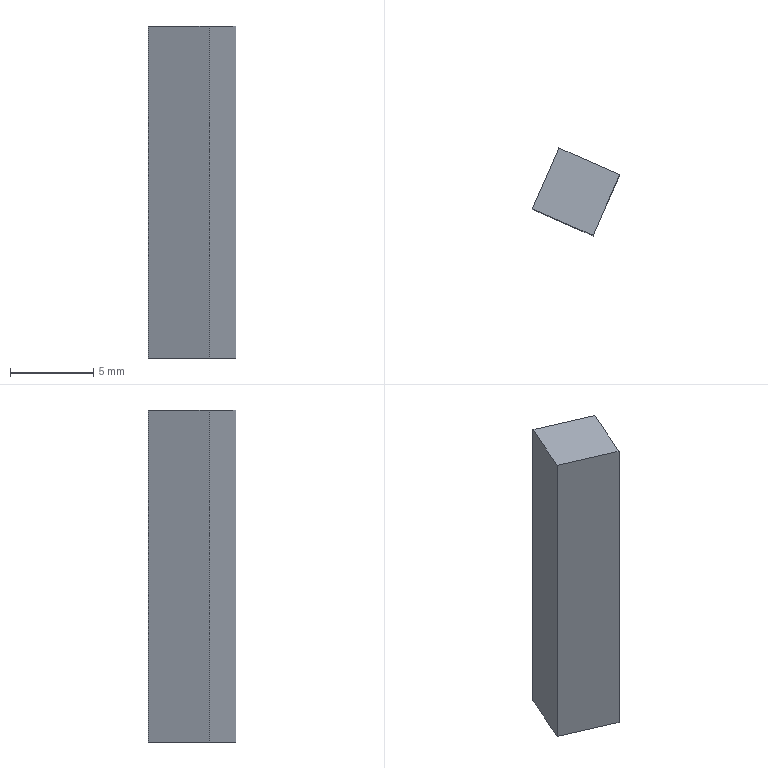Component | SolidWorks | 4X4FlatKey-1 | 1 solid | 6 faces | box 5.27 x 5.27 x 20 mm | volume 320 mm3 | plane 6
STEP:
#1=COLOUR_RGB('',0.7922,0.8196,0.9333);
#2=FILL_AREA_STYLE_COLOUR('',#1);
#3=FILL_AREA_STYLE('',(#2));
#4=SURFACE_STYLE_FILL_AREA(#3);
#5=SURFACE_SIDE_STYLE('',(#4));
#6=SURFACE_STYLE_USAGE(.BOTH.,#5);
#7=PRESENTATION_STYLE_ASSIGNMENT((#6));
#8=CARTESIAN_POINT('',(0.8561,0.498,4.6));
#9=VERTEX_POINT('',#8);
#10=CARTESIAN_POINT('',(1.,0.4349,4.6));
#11=VERTEX_POINT('',#10);
#12=CARTESIAN_POINT('',(0.8561,0.498,4.6));
#13=DIRECTION('',(0.9164,-0.4003,0.));
#14=VECTOR('',#13,39.37);
#15=LINE('',#12,#14);
#16=EDGE_CURVE('',#9,#11,#15,.T.);
#17=ORIENTED_EDGE('',*,*,#16,.T.);
#18=CARTESIAN_POINT('',(1.,0.4349,5.388));
#19=VERTEX_POINT('',#18);
#20=CARTESIAN_POINT('',(1.,0.4349,5.388));
#21=DIRECTION('',(0.,-0.,-1.));
#22=VECTOR('',#21,39.37);
#23=LINE('',#20,#22);
#24=EDGE_CURVE('',#19,#11,#23,.T.);
#25=ORIENTED_EDGE('',*,*,#24,.F.);
#26=CARTESIAN_POINT('',(0.8561,0.498,5.388));
#27=VERTEX_POINT('',#26);
#28=CARTESIAN_POINT('',(0.8561,0.498,5.388));
#29=DIRECTION('',(0.9164,-0.4003,0.));
#30=VECTOR('',#29,39.37);
#31=LINE('',#28,#30);
#32=EDGE_CURVE('',#27,#19,#31,.T.);
#33=ORIENTED_EDGE('',*,*,#32,.F.);
#34=CARTESIAN_POINT('',(0.8561,0.498,5.388));
#35=DIRECTION('',(0.,-0.,-1.));
#36=VECTOR('',#35,39.37);
#37=LINE('',#34,#36);
#38=EDGE_CURVE('',#27,#9,#37,.T.);
#39=ORIENTED_EDGE('',*,*,#38,.T.);
#40=EDGE_LOOP('',(#17,#25,#33,#39));
#41=FACE_OUTER_BOUND('',#40,.T.);
#42=CARTESIAN_POINT('',(0.8561,0.498,5.388));
#43=DIRECTION('',(0.4003,0.9164,0.));
#44=DIRECTION('',(0.,-0.,-1.));
#45=AXIS2_PLACEMENT_3D('',#42,#43,#44);
#46=PLANE('',#45);
#47=ADVANCED_FACE('',(#41),#46,.F.);
#48=CARTESIAN_POINT('',(1.063,0.5792,4.6));
#49=VERTEX_POINT('',#48);
#50=CARTESIAN_POINT('',(1.,0.4349,4.6));
#51=DIRECTION('',(0.4003,0.9164,0.));
#52=VECTOR('',#51,39.37);
#53=LINE('',#50,#52);
#54=EDGE_CURVE('',#11,#49,#53,.T.);
#55=ORIENTED_EDGE('',*,*,#54,.T.);
#56=CARTESIAN_POINT('',(1.063,0.5792,5.388));
#57=VERTEX_POINT('',#56);
#58=CARTESIAN_POINT('',(1.063,0.5792,5.388));
#59=DIRECTION('',(0.,-0.,-1.));
#60=VECTOR('',#59,39.37);
#61=LINE('',#58,#60);
#62=EDGE_CURVE('',#57,#49,#61,.T.);
#63=ORIENTED_EDGE('',*,*,#62,.F.);
#64=CARTESIAN_POINT('',(1.,0.4349,5.388));
#65=DIRECTION('',(0.4003,0.9164,0.));
#66=VECTOR('',#65,39.37);
#67=LINE('',#64,#66);
#68=EDGE_CURVE('',#19,#57,#67,.T.);
#69=ORIENTED_EDGE('',*,*,#68,.F.);
#70=ORIENTED_EDGE('',*,*,#24,.T.);
#71=EDGE_LOOP('',(#55,#63,#69,#70));
#72=FACE_OUTER_BOUND('',#71,.T.);
#73=CARTESIAN_POINT('',(1.,0.4349,5.388));
#74=DIRECTION('',(-0.9164,0.4003,-0.));
#75=DIRECTION('',(-0.,0.,1.));
#76=AXIS2_PLACEMENT_3D('',#73,#74,#75);
#77=PLANE('',#76);
#78=ADVANCED_FACE('',(#72),#77,.F.);
#79=CARTESIAN_POINT('',(0.9192,0.6423,4.6));
#80=VERTEX_POINT('',#79);
#81=CARTESIAN_POINT('',(0.9192,0.6423,4.6));
#82=DIRECTION('',(-0.9164,0.4003,-0.));
#83=VECTOR('',#82,39.37);
#84=LINE('',#81,#83);
#85=EDGE_CURVE('',#49,#80,#84,.T.);
#86=ORIENTED_EDGE('',*,*,#85,.T.);
#87=CARTESIAN_POINT('',(0.9192,0.6423,5.388));
#88=VERTEX_POINT('',#87);
#89=CARTESIAN_POINT('',(0.9192,0.6423,5.388));
#90=DIRECTION('',(0.,-0.,-1.));
#91=VECTOR('',#90,39.37);
#92=LINE('',#89,#91);
#93=EDGE_CURVE('',#88,#80,#92,.T.);
#94=ORIENTED_EDGE('',*,*,#93,.F.);
#95=CARTESIAN_POINT('',(0.9192,0.6423,5.388));
#96=DIRECTION('',(-0.9164,0.4003,-0.));
#97=VECTOR('',#96,39.37);
#98=LINE('',#95,#97);
#99=EDGE_CURVE('',#57,#88,#98,.T.);
#100=ORIENTED_EDGE('',*,*,#99,.F.);
#101=ORIENTED_EDGE('',*,*,#62,.T.);
#102=EDGE_LOOP('',(#86,#94,#100,#101));
#103=FACE_OUTER_BOUND('',#102,.T.);
#104=CARTESIAN_POINT('',(0.9192,0.6423,5.388));
#105=DIRECTION('',(-0.4003,-0.9164,-0.));
#106=DIRECTION('',(0.9164,-0.4003,0.));
#107=AXIS2_PLACEMENT_3D('',#104,#105,#106);
#108=PLANE('',#107);
#109=ADVANCED_FACE('',(#103),#108,.F.);
#110=CARTESIAN_POINT('',(0.8561,0.498,4.6));
#111=DIRECTION('',(-0.4003,-0.9164,-0.));
#112=VECTOR('',#111,39.37);
#113=LINE('',#110,#112);
#114=EDGE_CURVE('',#80,#9,#113,.T.);
#115=ORIENTED_EDGE('',*,*,#114,.T.);
#116=ORIENTED_EDGE('',*,*,#38,.F.);
#117=CARTESIAN_POINT('',(0.8561,0.498,5.388));
#118=DIRECTION('',(-0.4003,-0.9164,-0.));
#119=VECTOR('',#118,39.37);
#120=LINE('',#117,#119);
#121=EDGE_CURVE('',#88,#27,#120,.T.);
#122=ORIENTED_EDGE('',*,*,#121,.F.);
#123=ORIENTED_EDGE('',*,*,#93,.T.);
#124=EDGE_LOOP('',(#115,#116,#122,#123));
#125=FACE_OUTER_BOUND('',#124,.T.);
#126=CARTESIAN_POINT('',(0.8561,0.498,5.388));
#127=DIRECTION('',(0.9164,-0.4003,0.));
#128=DIRECTION('',(0.,-0.,-1.));
#129=AXIS2_PLACEMENT_3D('',#126,#127,#128);
#130=PLANE('',#129);
#131=ADVANCED_FACE('',(#125),#130,.F.);
#132=ORIENTED_EDGE('',*,*,#32,.T.);
#133=ORIENTED_EDGE('',*,*,#68,.T.);
#134=ORIENTED_EDGE('',*,*,#99,.T.);
#135=ORIENTED_EDGE('',*,*,#121,.T.);
#136=EDGE_LOOP('',(#132,#133,#134,#135));
#137=FACE_OUTER_BOUND('',#136,.T.);
#138=CARTESIAN_POINT('',(0.7581,1.021,5.388));
#139=DIRECTION('',(-0.,0.,1.));
#140=DIRECTION('',(0.4003,0.9164,0.));
#141=AXIS2_PLACEMENT_3D('',#138,#139,#140);
#142=PLANE('',#141);
#143=ADVANCED_FACE('',(#137),#142,.T.);
#144=ORIENTED_EDGE('',*,*,#16,.F.);
#145=ORIENTED_EDGE('',*,*,#114,.F.);
#146=ORIENTED_EDGE('',*,*,#85,.F.);
#147=ORIENTED_EDGE('',*,*,#54,.F.);
#148=EDGE_LOOP('',(#144,#145,#146,#147));
#149=FACE_OUTER_BOUND('',#148,.T.);
#150=CARTESIAN_POINT('',(0.7581,1.021,4.6));
#151=DIRECTION('',(-0.,0.,1.));
#152=DIRECTION('',(0.4003,0.9164,0.));
#153=AXIS2_PLACEMENT_3D('',#150,#151,#152);
#154=PLANE('',#153);
#155=ADVANCED_FACE('',(#149),#154,.F.);
#156=CLOSED_SHELL('',(#47,#78,#109,#131,#143,#155));
#157=MANIFOLD_SOLID_BREP('',#156);
#158=STYLED_ITEM('',(#7),#157);
#159=(LENGTH_UNIT()NAMED_UNIT(*)SI_UNIT($,.METRE.));
#160=LENGTH_MEASURE_WITH_UNIT(LENGTH_MEASURE(0.0254),#159);
#161=DIMENSIONAL_EXPONENTS(1.,0.,0.,0.,0.,0.,0.);
#162=(CONVERSION_BASED_UNIT('',#160)LENGTH_UNIT()NAMED_UNIT(#161));
#163=UNCERTAINTY_MEASURE_WITH_UNIT(LENGTH_MEASURE(0.00001),#162,'','');
#164=(NAMED_UNIT(*)PLANE_ANGLE_UNIT()SI_UNIT($,.RADIAN.));
#165=(NAMED_UNIT(*)SI_UNIT($,.STERADIAN.)SOLID_ANGLE_UNIT());
#166=(GEOMETRIC_REPRESENTATION_CONTEXT(3)GLOBAL_UNCERTAINTY_ASSIGNED_CONTEXT((#163))GLOBAL_UNIT_ASSIGNED_CONTEXT((#162,#164,#165))REPRESENTATION_CONTEXT('',''));
#167=MECHANICAL_DESIGN_GEOMETRIC_PRESENTATION_REPRESENTATION('',(#158),#166);
#168=CARTESIAN_POINT('',(0.,0.,0.));
#169=DIRECTION('',(0.,0.,1.));
#170=DIRECTION('',(1.,0.,0.));
#171=AXIS2_PLACEMENT_3D('',#168,#169,#170);
#172=(LENGTH_UNIT()NAMED_UNIT(*)SI_UNIT($,.METRE.));
#173=LENGTH_MEASURE_WITH_UNIT(LENGTH_MEASURE(0.0254),#172);
#174=DIMENSIONAL_EXPONENTS(1.,0.,0.,0.,0.,0.,0.);
#175=(CONVERSION_BASED_UNIT('',#173)LENGTH_UNIT()NAMED_UNIT(#174));
#176=UNCERTAINTY_MEASURE_WITH_UNIT(LENGTH_MEASURE(0.00001),#175,'','');
#177=(NAMED_UNIT(*)PLANE_ANGLE_UNIT()SI_UNIT($,.RADIAN.));
#178=(NAMED_UNIT(*)SI_UNIT($,.STERADIAN.)SOLID_ANGLE_UNIT());
#179=(GEOMETRIC_REPRESENTATION_CONTEXT(3)GLOBAL_UNCERTAINTY_ASSIGNED_CONTEXT((#176))GLOBAL_UNIT_ASSIGNED_CONTEXT((#175,#177,#178))REPRESENTATION_CONTEXT('',''));
#180=ADVANCED_BREP_SHAPE_REPRESENTATION('',(#157,#171),#179);
#181=PRESENTATION_LAYER_ASSIGNMENT('','',(#158));